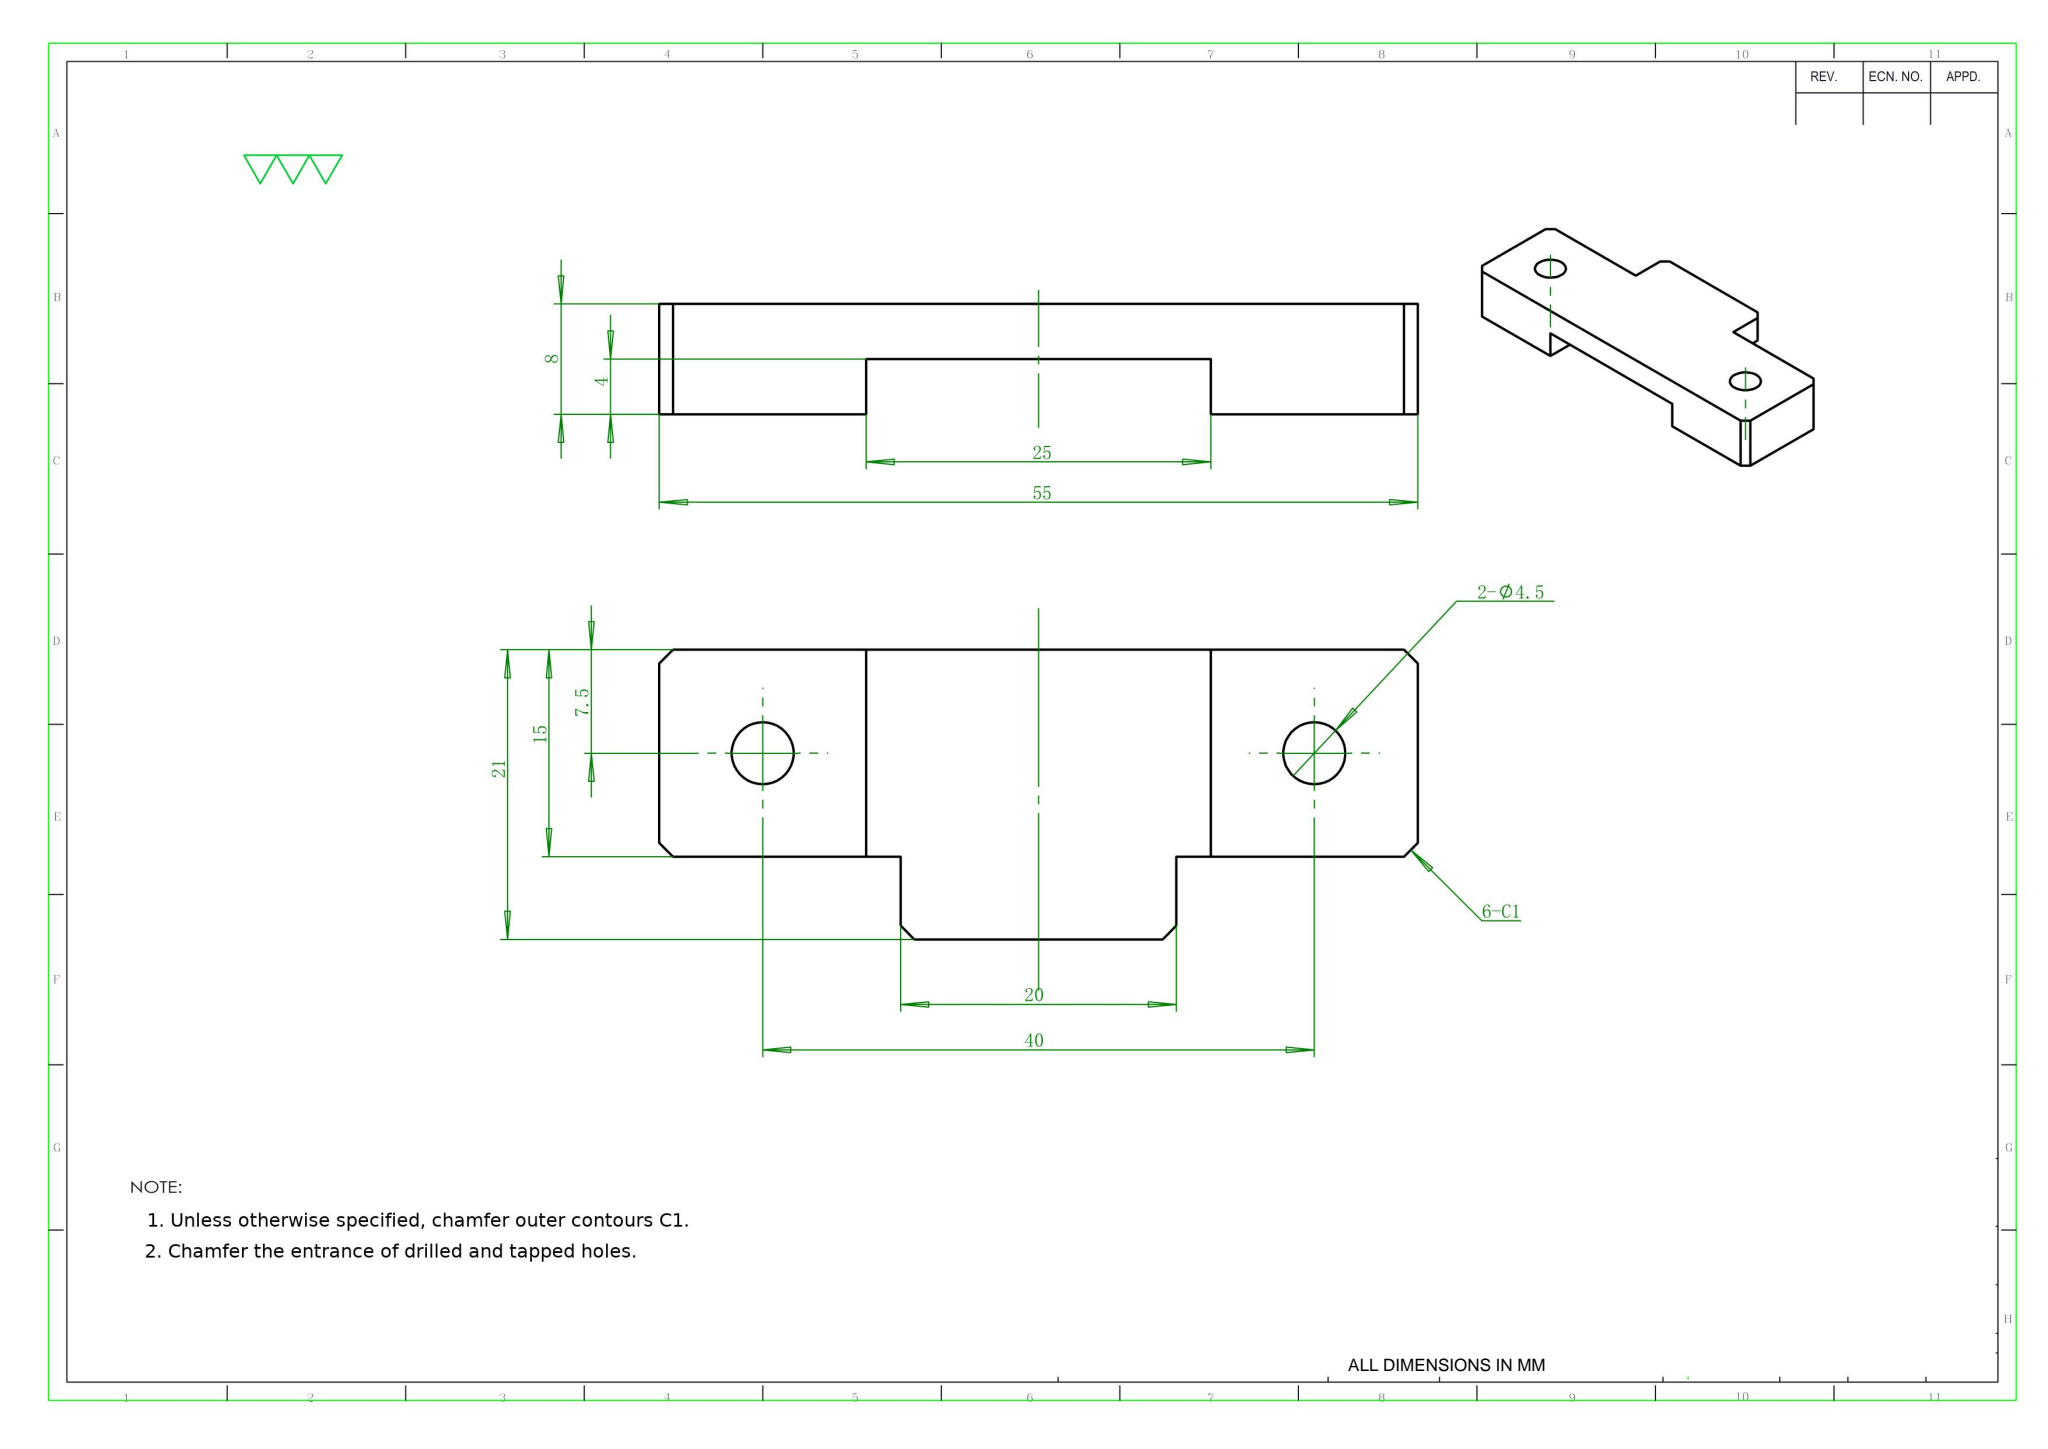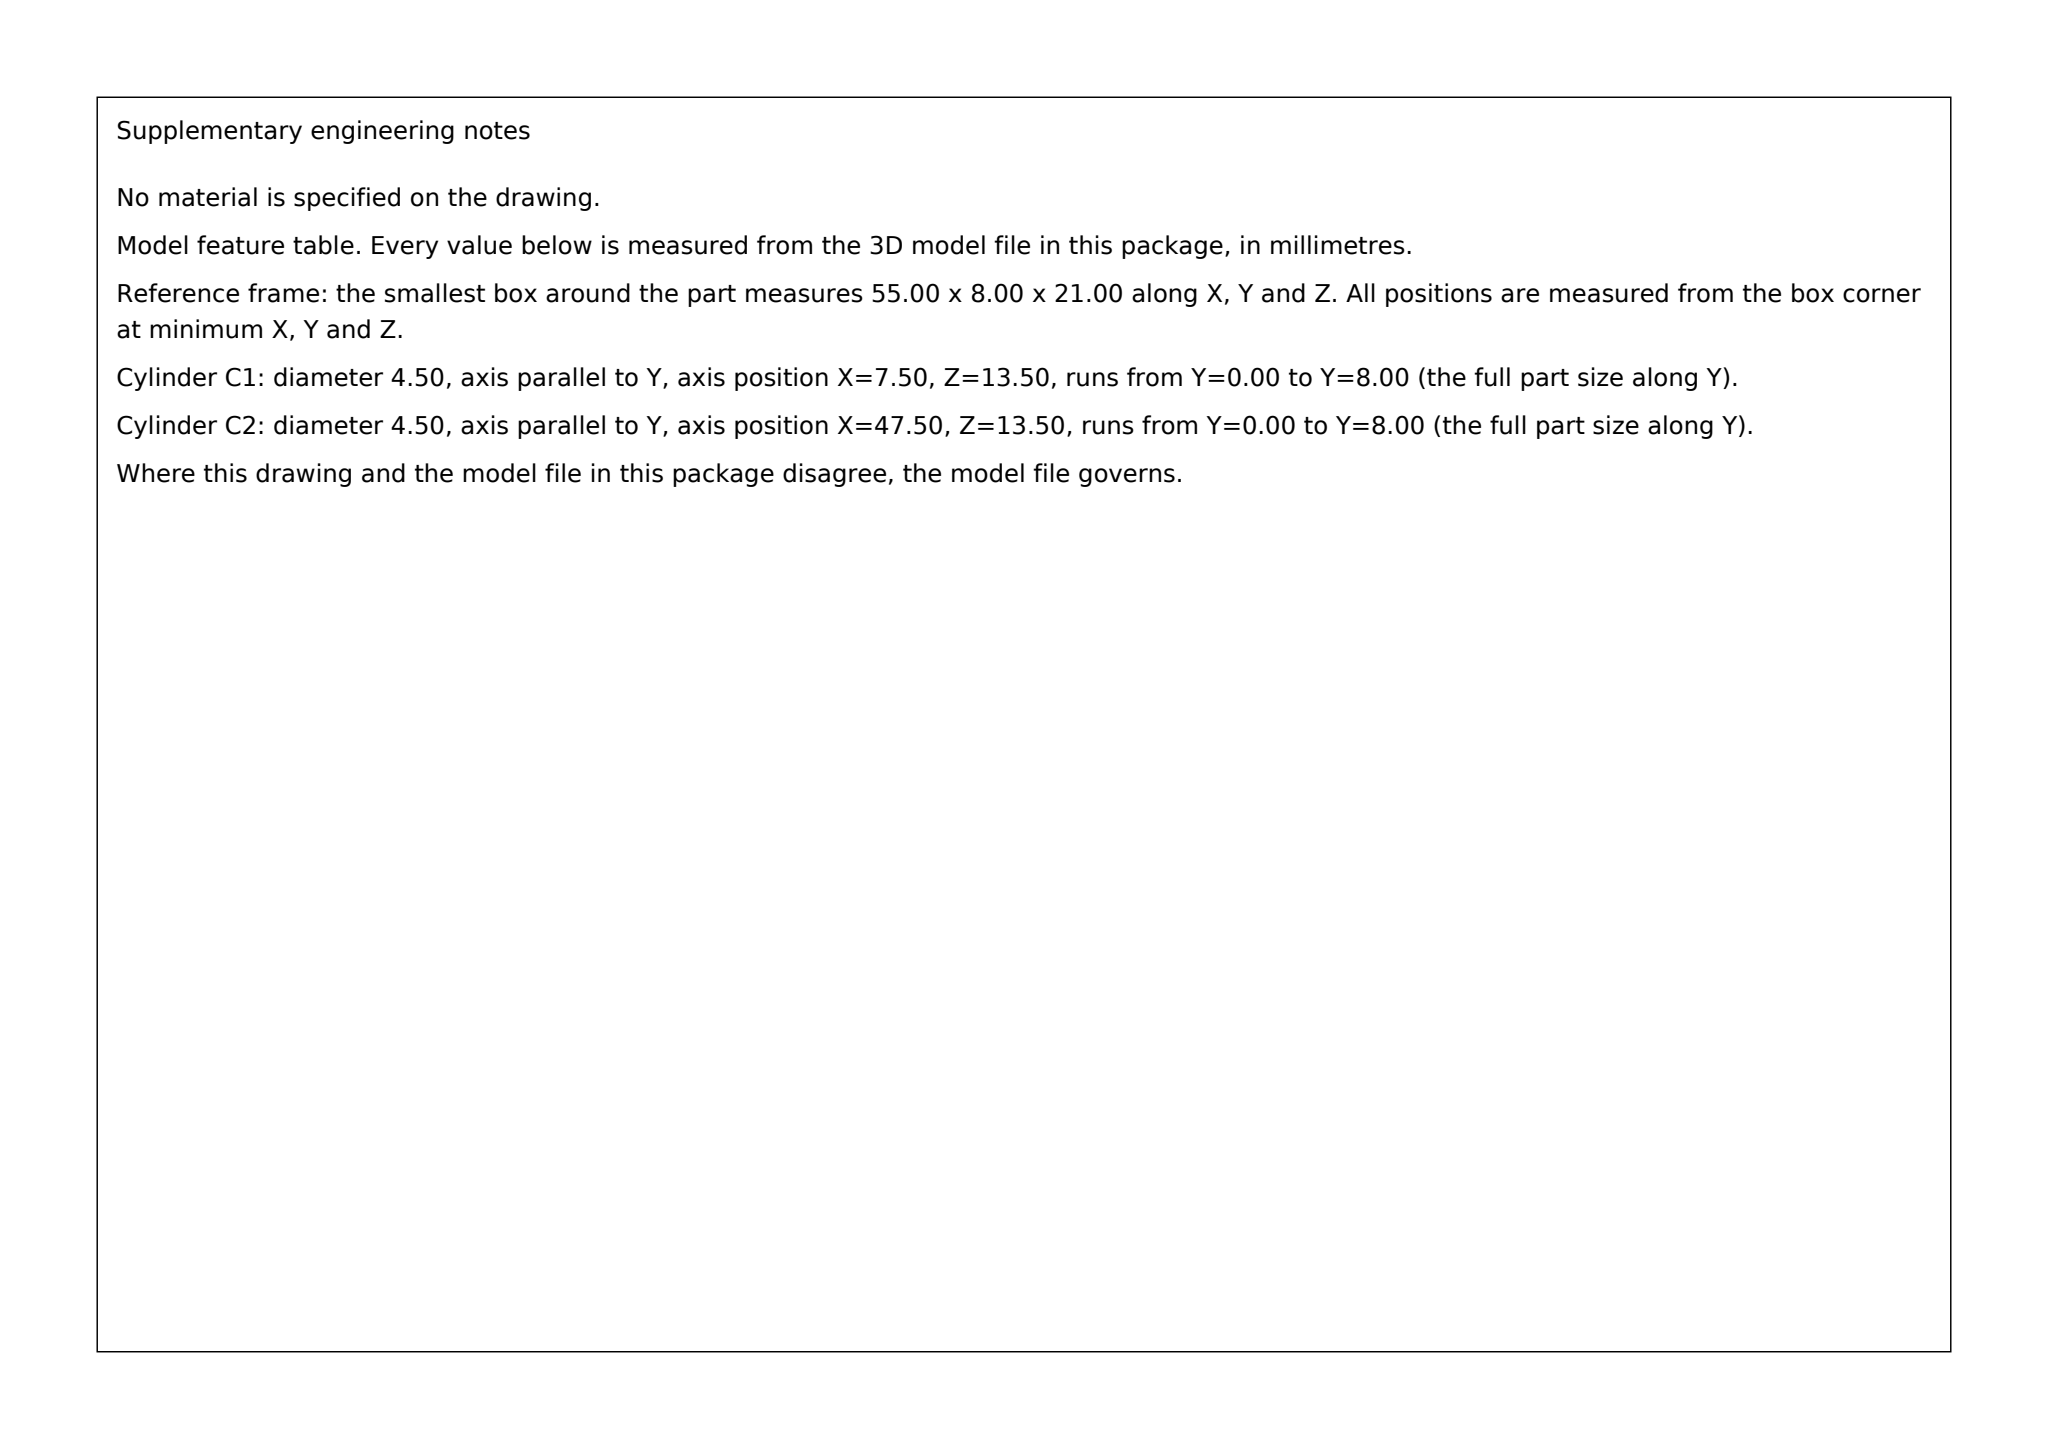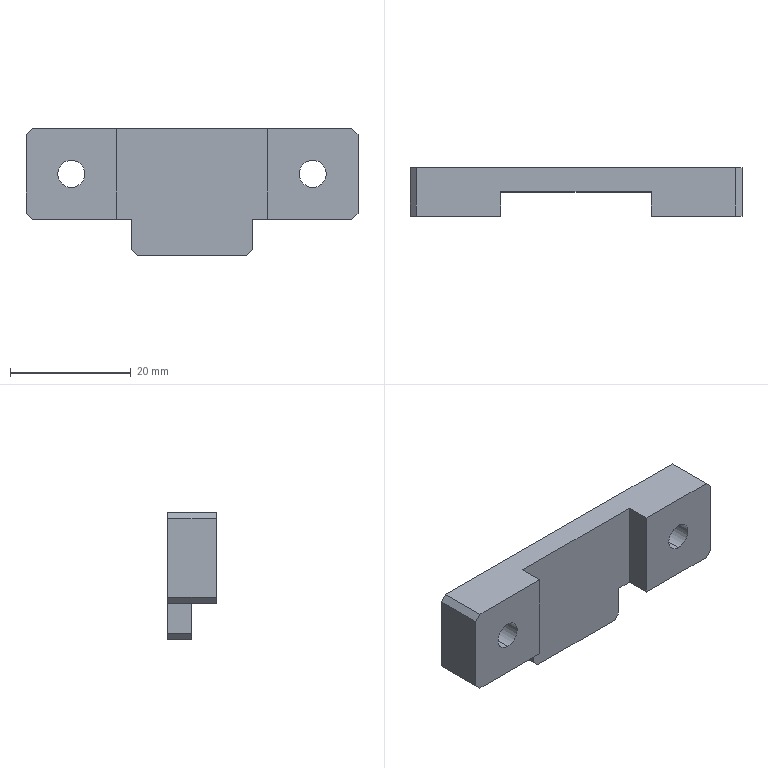Part | SolidWorks | mm | 1 solid | 24 faces | box 55 x 8 x 21 mm | volume 5306 mm3 | plane 20 | cylinder 4 | commonest cylinder face diameters 4.5 x4
build123d program:
from build123d import *

# Parameters (mm, degrees)
BOSS_EXTRUDE1_DEPTH        = 8
SKETCH2_W                  = 25
SKETCH2_H                  = 4
CUT_EXTRUDE1_DEPTH         = 36.514
F_4_5_4_5_DIAMETER_HOLE1_D = 4.5
CHAMFER1_SIZE              = 1


with BuildPart() as part:
    # Sketch1 → Boss-Extrude1 (new body)
    with BuildSketch(Plane(origin=(0, 0, 0), x_dir=(1, 0, 0), z_dir=(0, 1, 0))):
        Polygon((-27.5, 0), (-27.5, 15), (-10, 15), (-10, 21), (10, 21), (10, 15), (27.5, 15), (27.5, 0), align=None)
    extrude(amount=BOSS_EXTRUDE1_DEPTH)

    # Sketch2 → Cut-Extrude1 (cut, through all)
    with BuildSketch(Plane.XY):
        with Locations((0, 2)):
            Rectangle(SKETCH2_W, SKETCH2_H)
    extrude(amount=-CUT_EXTRUDE1_DEPTH, mode=Mode.SUBTRACT)

    # 4.5 _4.5_ Diameter Hole1 (through all)
    with Locations(Plane(origin=(0, 8, 0), x_dir=(1, 0, 0), z_dir=(0, 1, 0))):
        with Locations((20, 7.5), (-20, 7.5)):
            Hole(F_4_5_4_5_DIAMETER_HOLE1_D / 2)

    # Chamfer1
    chamfer1_edges = [part.edges().sort_by_distance(p)[0] for p in [
        (-27.5, 4, 0),
        (-27.5, 4, -15),
        (-10, 6, -21),
        (10, 6, -21),
        (27.5, 4, -15),
        (27.5, 4, 0),
    ]]
    chamfer(chamfer1_edges, length=CHAMFER1_SIZE)


solid = part.part